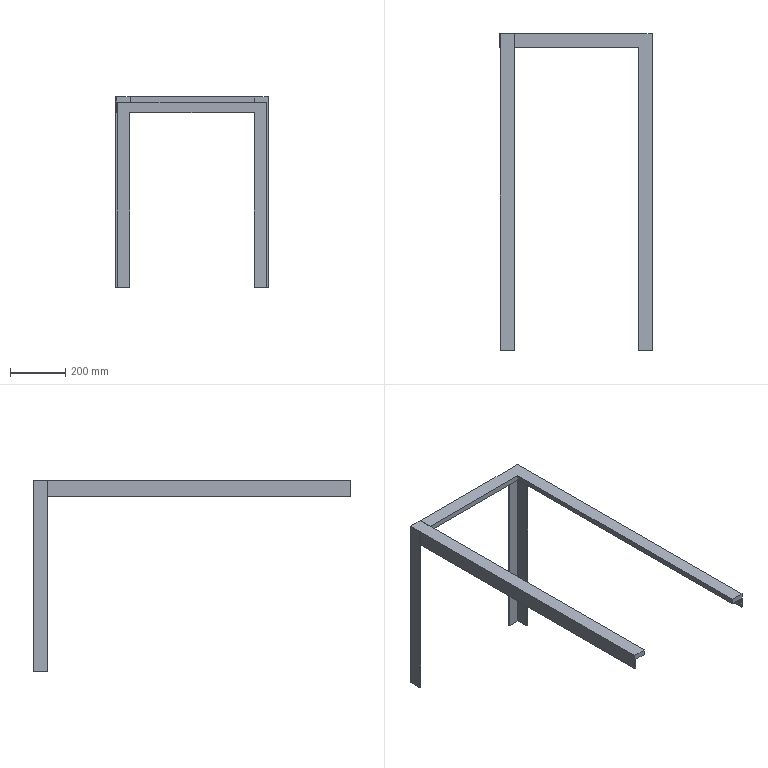Component | NX | REAR_SUPPORT_BRACKET | 1 solid | 33 faces | volume 3883129 mm3 | plane 33